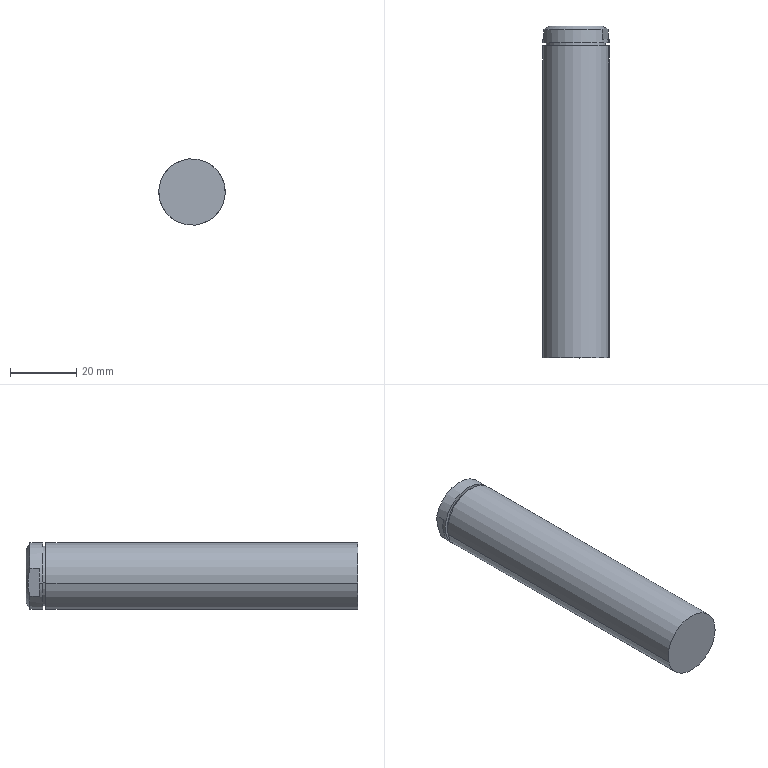Component | SolidWorks | SDA50-80CylinderPiston-1 | 1 solid | 20 faces | box 20 x 100 x 20 mm | volume 29602 mm3 | cylinder 8 | plane 8 | cone 4 | commonest cylinder face diameters 20 x4 18 x2 8.8 x2
build123d program:
from build123d import *

# Parameters (mm, degrees)
SKETCH1_R                   = 10
BOSS_EXTRUDE1_DEPTH         = 100
CHAMFER1_SIZE               = 2
CHAMFER1_SIZE2              = 1.155
CUT_EXTRUDE2_DEPTH          = 4
M10X1_25_TAPPED_HOLE1_D     = 8.8
M10X1_25_TAPPED_HOLE1_DEPTH = 26.25
M10X1_25_TAPPED_HOLE1_TIP   = 2.644
SKETCH6_W                   = 1
SKETCH6_H                   = 1


with BuildPart() as part:
    # Sketch1 → Boss-Extrude1 (new body)
    with BuildSketch(Plane.XY):
        Circle(SKETCH1_R)
    extrude(amount=BOSS_EXTRUDE1_DEPTH)

    # Chamfer1
    chamfer1_edges = [part.edges().sort_by_distance(p)[0] for p in [
        (-10, 0, 0),
    ]]
    chamfer1_side = [part.faces().sort_by_distance(p)[0] for p in [
        (0, 0, 0),
    ]]
    chamfer(chamfer1_edges, length=CHAMFER1_SIZE, length2=CHAMFER1_SIZE2, reference=chamfer1_side[0])

    # Sketch3 → Cut-Extrude2 (cut)
    with BuildSketch(Plane(origin=(0, 0, 0), x_dir=(-1, 0, 0), z_dir=(0, 0, -1))):
        with BuildLine():
            Line((9, 4.359), (9, -4.359))
            ThreePointArc((9, -4.359), (10, 0), (9, 4.359))
        make_face()
        with BuildLine():
            Line((-9, 4.359), (-9, -4.359))
            ThreePointArc((-9, -4.359), (-10, 0), (-9, 4.359))
        make_face()
    extrude(amount=-CUT_EXTRUDE2_DEPTH, mode=Mode.SUBTRACT)

    # M10x1.25 Tapped Hole1
    with Locations(Plane(origin=(0, 0, 0), x_dir=(-1, 0, 0), z_dir=(0, 0, -1))):
        with Locations((0, 0)):
            Hole(M10X1_25_TAPPED_HOLE1_D / 2, depth=M10X1_25_TAPPED_HOLE1_DEPTH)
            with Locations((0, 0, -(M10X1_25_TAPPED_HOLE1_DEPTH + M10X1_25_TAPPED_HOLE1_TIP / 2))):  # 118° drill point
                Cone(0, M10X1_25_TAPPED_HOLE1_D / 2, M10X1_25_TAPPED_HOLE1_TIP, mode=Mode.SUBTRACT)

    # Sketch6 → Cut-Revolve3 (revolve, cut)
    with BuildSketch(Plane(origin=(0, 0, 0), x_dir=(1, 0, 0), z_dir=(0, 1, 0))):
        with Locations((-9.5, -5.5)):
            Rectangle(SKETCH6_W, SKETCH6_H)
    revolve(axis=Axis((0, 0, 0), (0, 0, 1)), mode=Mode.SUBTRACT)


solid = part.part

# Placed as in the assembly
solid = solid.moved(Location((-29.507, -49.411, 430.5), (90, 0, 12.223)))
STEP:
#1=CARTESIAN_POINT('',(-0.7769,-5.882,17.032));
#2=VERTEX_POINT('',#1);
#3=CARTESIAN_POINT('',(-1.546,-5.882,16.865));
#4=VERTEX_POINT('',#3);
#5=CARTESIAN_POINT('',(-1.162,-5.882,16.949));
#6=DIRECTION('',(0.,-1.,0.));
#7=DIRECTION('',(0.9773,0.,0.2117));
#8=AXIS2_PLACEMENT_3D('',#5,#6,#7);
#9=CIRCLE('',#8,0.3937);
#10=EDGE_CURVE('',#2,#4,#9,.T.);
#11=ORIENTED_EDGE('',*,*,#10,.F.);
#12=CARTESIAN_POINT('',(-0.7769,-2.182,17.032));
#13=VERTEX_POINT('',#12);
#14=CARTESIAN_POINT('',(-0.7769,-5.882,17.032));
#15=DIRECTION('',(-0.,1.,-0.));
#16=VECTOR('',#15,39.37);
#17=LINE('',#14,#16);
#18=EDGE_CURVE('',#2,#13,#17,.T.);
#19=ORIENTED_EDGE('',*,*,#18,.T.);
#20=CARTESIAN_POINT('',(-1.546,-2.182,16.865));
#21=VERTEX_POINT('',#20);
#22=CARTESIAN_POINT('',(-1.162,-2.182,16.949));
#23=DIRECTION('',(-0.,1.,-0.));
#24=DIRECTION('',(-0.9773,0.,-0.2117));
#25=AXIS2_PLACEMENT_3D('',#22,#23,#24);
#26=CIRCLE('',#25,0.3937);
#27=EDGE_CURVE('',#21,#13,#26,.T.);
#28=ORIENTED_EDGE('',*,*,#27,.F.);
#29=CARTESIAN_POINT('',(-1.546,-5.882,16.865));
#30=DIRECTION('',(-0.,1.,-0.));
#31=VECTOR('',#30,39.37);
#32=LINE('',#29,#31);
#33=EDGE_CURVE('',#4,#21,#32,.T.);
#34=ORIENTED_EDGE('',*,*,#33,.F.);
#35=EDGE_LOOP('',(#11,#19,#28,#34));
#36=FACE_OUTER_BOUND('',#35,.T.);
#37=CARTESIAN_POINT('',(-1.162,-5.882,16.949));
#38=DIRECTION('',(-0.,1.,-0.));
#39=DIRECTION('',(-0.9773,0.,-0.2117));
#40=AXIS2_PLACEMENT_3D('',#37,#38,#39);
#41=CYLINDRICAL_SURFACE('',#40,0.3937);
#42=ADVANCED_FACE('',(#36),#41,.T.);
#43=CARTESIAN_POINT('',(-1.508,-2.182,16.874));
#44=VERTEX_POINT('',#43);
#45=CARTESIAN_POINT('',(-0.8154,-2.182,17.024));
#46=VERTEX_POINT('',#45);
#47=CARTESIAN_POINT('',(-1.162,-2.182,16.949));
#48=DIRECTION('',(-0.,1.,-0.));
#49=DIRECTION('',(-0.9773,0.,-0.2117));
#50=AXIS2_PLACEMENT_3D('',#47,#48,#49);
#51=CIRCLE('',#50,0.3543);
#52=EDGE_CURVE('',#44,#46,#51,.T.);
#53=ORIENTED_EDGE('',*,*,#52,.T.);
#54=CARTESIAN_POINT('',(-0.8154,-2.142,17.024));
#55=VERTEX_POINT('',#54);
#56=CARTESIAN_POINT('',(-0.8154,-1.945,17.024));
#57=DIRECTION('',(-0.,1.,-0.));
#58=VECTOR('',#57,39.37);
#59=LINE('',#56,#58);
#60=EDGE_CURVE('',#46,#55,#59,.T.);
#61=ORIENTED_EDGE('',*,*,#60,.T.);
#62=CARTESIAN_POINT('',(-1.508,-2.142,16.874));
#63=VERTEX_POINT('',#62);
#64=CARTESIAN_POINT('',(-1.162,-2.142,16.949));
#65=DIRECTION('',(-0.,1.,-0.));
#66=DIRECTION('',(-0.9773,0.,-0.2117));
#67=AXIS2_PLACEMENT_3D('',#64,#65,#66);
#68=CIRCLE('',#67,0.3543);
#69=EDGE_CURVE('',#63,#55,#68,.T.);
#70=ORIENTED_EDGE('',*,*,#69,.F.);
#71=CARTESIAN_POINT('',(-1.508,-1.945,16.874));
#72=DIRECTION('',(-0.,1.,-0.));
#73=VECTOR('',#72,39.37);
#74=LINE('',#71,#73);
#75=EDGE_CURVE('',#44,#63,#74,.T.);
#76=ORIENTED_EDGE('',*,*,#75,.F.);
#77=EDGE_LOOP('',(#53,#61,#70,#76));
#78=FACE_OUTER_BOUND('',#77,.T.);
#79=CARTESIAN_POINT('',(-1.162,-1.945,16.949));
#80=DIRECTION('',(-0.,1.,-0.));
#81=DIRECTION('',(-0.9773,0.,-0.2117));
#82=AXIS2_PLACEMENT_3D('',#79,#80,#81);
#83=CYLINDRICAL_SURFACE('',#82,0.3543);
#84=ADVANCED_FACE('',(#78),#83,.T.);
#85=CARTESIAN_POINT('',(-0.9924,-2.979,16.985));
#86=VERTEX_POINT('',#85);
#87=CARTESIAN_POINT('',(-1.331,-2.979,16.912));
#88=VERTEX_POINT('',#87);
#89=CARTESIAN_POINT('',(-1.162,-2.979,16.949));
#90=DIRECTION('',(-0.,1.,-0.));
#91=DIRECTION('',(-0.9773,0.,-0.2117));
#92=AXIS2_PLACEMENT_3D('',#89,#90,#91);
#93=CIRCLE('',#92,0.1732);
#94=EDGE_CURVE('',#86,#88,#93,.T.);
#95=ORIENTED_EDGE('',*,*,#94,.F.);
#96=CARTESIAN_POINT('',(-0.9924,-1.945,16.985));
#97=VERTEX_POINT('',#96);
#98=CARTESIAN_POINT('',(-0.9924,-1.945,16.985));
#99=DIRECTION('',(-0.,1.,-0.));
#100=VECTOR('',#99,39.37);
#101=LINE('',#98,#100);
#102=EDGE_CURVE('',#86,#97,#101,.T.);
#103=ORIENTED_EDGE('',*,*,#102,.T.);
#104=CARTESIAN_POINT('',(-1.331,-1.945,16.912));
#105=VERTEX_POINT('',#104);
#106=CARTESIAN_POINT('',(-1.162,-1.945,16.949));
#107=DIRECTION('',(-0.,1.,-0.));
#108=DIRECTION('',(-0.9773,0.,-0.2117));
#109=AXIS2_PLACEMENT_3D('',#106,#107,#108);
#110=CIRCLE('',#109,0.1732);
#111=EDGE_CURVE('',#97,#105,#110,.T.);
#112=ORIENTED_EDGE('',*,*,#111,.T.);
#113=CARTESIAN_POINT('',(-1.331,-1.945,16.912));
#114=DIRECTION('',(-0.,1.,-0.));
#115=VECTOR('',#114,39.37);
#116=LINE('',#113,#115);
#117=EDGE_CURVE('',#88,#105,#116,.T.);
#118=ORIENTED_EDGE('',*,*,#117,.F.);
#119=EDGE_LOOP('',(#95,#103,#112,#118));
#120=FACE_OUTER_BOUND('',#119,.T.);
#121=CARTESIAN_POINT('',(-1.162,-1.945,16.949));
#122=DIRECTION('',(-0.,1.,-0.));
#123=DIRECTION('',(-0.9773,0.,-0.2117));
#124=AXIS2_PLACEMENT_3D('',#121,#122,#123);
#125=CYLINDRICAL_SURFACE('',#124,0.1732);
#126=ADVANCED_FACE('',(#120),#125,.F.);
#127=CARTESIAN_POINT('',(-1.162,-3.083,16.949));
#128=VERTEX_POINT('',#127);
#129=CARTESIAN_POINT('',(-1.331,-2.979,16.912));
#130=DIRECTION('',(-0.8377,0.515,-0.1815));
#131=VECTOR('',#130,39.37);
#132=LINE('',#129,#131);
#133=EDGE_CURVE('',#128,#88,#132,.T.);
#134=ORIENTED_EDGE('',*,*,#133,.F.);
#135=CARTESIAN_POINT('',(-0.9924,-2.979,16.985));
#136=DIRECTION('',(0.8377,0.515,0.1815));
#137=VECTOR('',#136,39.37);
#138=LINE('',#135,#137);
#139=EDGE_CURVE('',#128,#86,#138,.T.);
#140=ORIENTED_EDGE('',*,*,#139,.T.);
#141=ORIENTED_EDGE('',*,*,#94,.T.);
#142=EDGE_LOOP('',(#134,#140,#141));
#143=FACE_OUTER_BOUND('',#142,.T.);
#144=CARTESIAN_POINT('',(-1.162,-2.979,16.949));
#145=DIRECTION('',(-0.,1.,-0.));
#146=DIRECTION('',(-0.9773,0.,-0.2117));
#147=AXIS2_PLACEMENT_3D('',#144,#145,#146);
#148=CONICAL_SURFACE('',#147,0.1732,1.03);
#149=ADVANCED_FACE('',(#143),#148,.F.);
#150=CARTESIAN_POINT('',(-1.469,-1.945,16.882));
#151=VERTEX_POINT('',#150);
#152=CARTESIAN_POINT('',(-0.8539,-1.945,17.016));
#153=VERTEX_POINT('',#152);
#154=CARTESIAN_POINT('',(-1.162,-1.945,16.949));
#155=DIRECTION('',(-0.,1.,-0.));
#156=DIRECTION('',(0.9773,0.,0.2117));
#157=AXIS2_PLACEMENT_3D('',#154,#155,#156);
#158=CIRCLE('',#157,0.315);
#159=EDGE_CURVE('',#151,#153,#158,.T.);
#160=ORIENTED_EDGE('',*,*,#159,.F.);
#161=CARTESIAN_POINT('',(-1.508,-1.968,16.874));
#162=VERTEX_POINT('',#161);
#163=CARTESIAN_POINT('',(-1.546,-1.991,16.865));
#164=DIRECTION('',(-0.8464,-0.5,-0.1834));
#165=VECTOR('',#164,39.37);
#166=LINE('',#163,#165);
#167=EDGE_CURVE('',#151,#162,#166,.T.);
#168=ORIENTED_EDGE('',*,*,#167,.T.);
#169=CARTESIAN_POINT('',(-1.544,-1.991,17.042));
#170=VERTEX_POINT('',#169);
#171=CARTESIAN_POINT('',(-1.544,-1.991,17.042));
#172=CARTESIAN_POINT('',(-1.538,-1.984,17.014));
#173=CARTESIAN_POINT('',(-1.532,-1.978,16.987));
#174=CARTESIAN_POINT('',(-1.523,-1.972,16.944));
#175=CARTESIAN_POINT('',(-1.52,-1.971,16.93));
#176=CARTESIAN_POINT('',(-1.514,-1.969,16.902));
#177=CARTESIAN_POINT('',(-1.511,-1.968,16.888));
#178=CARTESIAN_POINT('',(-1.508,-1.968,16.874));
#179=B_SPLINE_CURVE_WITH_KNOTS('',3,(#171,#172,#173,#174,#175,#176,#177,#178),.UNSPECIFIED.,.F.,.F.,(4,2,2,4),(0.005779,0.007969,0.009064,0.01016),.UNSPECIFIED.);
#180=EDGE_CURVE('',#170,#162,#179,.T.);
#181=ORIENTED_EDGE('',*,*,#180,.F.);
#182=CARTESIAN_POINT('',(-0.8517,-1.991,17.192));
#183=VERTEX_POINT('',#182);
#184=CARTESIAN_POINT('',(-1.162,-1.991,16.949));
#185=DIRECTION('',(0.,-1.,0.));
#186=DIRECTION('',(0.9773,0.,0.2117));
#187=AXIS2_PLACEMENT_3D('',#184,#185,#186);
#188=CIRCLE('',#187,0.3937);
#189=EDGE_CURVE('',#183,#170,#188,.T.);
#190=ORIENTED_EDGE('',*,*,#189,.F.);
#191=CARTESIAN_POINT('',(-0.8154,-1.968,17.024));
#192=VERTEX_POINT('',#191);
#193=CARTESIAN_POINT('',(-0.8154,-1.968,17.024));
#194=CARTESIAN_POINT('',(-0.8184,-1.968,17.038));
#195=CARTESIAN_POINT('',(-0.8215,-1.969,17.052));
#196=CARTESIAN_POINT('',(-0.8276,-1.971,17.08));
#197=CARTESIAN_POINT('',(-0.8307,-1.972,17.094));
#198=CARTESIAN_POINT('',(-0.8398,-1.978,17.137));
#199=CARTESIAN_POINT('',(-0.8458,-1.984,17.164));
#200=CARTESIAN_POINT('',(-0.8517,-1.991,17.192));
#201=B_SPLINE_CURVE_WITH_KNOTS('',3,(#193,#194,#195,#196,#197,#198,#199,#200),.UNSPECIFIED.,.F.,.F.,(4,2,2,4),(0.01291,0.014,0.0151,0.01729),.UNSPECIFIED.);
#202=EDGE_CURVE('',#192,#183,#201,.T.);
#203=ORIENTED_EDGE('',*,*,#202,.F.);
#204=CARTESIAN_POINT('',(-0.7769,-1.991,17.032));
#205=DIRECTION('',(0.8464,-0.5,0.1834));
#206=VECTOR('',#205,39.37);
#207=LINE('',#204,#206);
#208=EDGE_CURVE('',#153,#192,#207,.T.);
#209=ORIENTED_EDGE('',*,*,#208,.F.);
#210=EDGE_LOOP('',(#160,#168,#181,#190,#203,#209));
#211=FACE_OUTER_BOUND('',#210,.T.);
#212=CARTESIAN_POINT('',(-1.162,-1.991,16.949));
#213=DIRECTION('',(0.,-1.,0.));
#214=DIRECTION('',(0.9773,0.,0.2117));
#215=AXIS2_PLACEMENT_3D('',#212,#213,#214);
#216=CONICAL_SURFACE('',#215,0.3937,1.047);
#217=ADVANCED_FACE('',(#211),#216,.T.);
#218=CARTESIAN_POINT('',(-1.546,-2.142,16.865));
#219=VERTEX_POINT('',#218);
#220=CARTESIAN_POINT('',(-0.7769,-2.142,17.032));
#221=VERTEX_POINT('',#220);
#222=CARTESIAN_POINT('',(-1.162,-2.142,16.949));
#223=DIRECTION('',(-0.,1.,-0.));
#224=DIRECTION('',(-0.9773,0.,-0.2117));
#225=AXIS2_PLACEMENT_3D('',#222,#223,#224);
#226=CIRCLE('',#225,0.3937);
#227=EDGE_CURVE('',#219,#221,#226,.T.);
#228=ORIENTED_EDGE('',*,*,#227,.T.);
#229=CARTESIAN_POINT('',(-0.7769,-2.103,17.032));
#230=VERTEX_POINT('',#229);
#231=CARTESIAN_POINT('',(-0.7769,-5.882,17.032));
#232=DIRECTION('',(-0.,1.,-0.));
#233=VECTOR('',#232,39.37);
#234=LINE('',#231,#233);
#235=EDGE_CURVE('',#221,#230,#234,.T.);
#236=ORIENTED_EDGE('',*,*,#235,.T.);
#237=CARTESIAN_POINT('',(-0.8517,-2.103,17.192));
#238=VERTEX_POINT('',#237);
#239=CARTESIAN_POINT('',(-1.162,-2.103,16.949));
#240=DIRECTION('',(-0.,1.,-0.));
#241=DIRECTION('',(-0.9773,0.,-0.2117));
#242=AXIS2_PLACEMENT_3D('',#239,#240,#241);
#243=CIRCLE('',#242,0.3937);
#244=EDGE_CURVE('',#238,#230,#243,.T.);
#245=ORIENTED_EDGE('',*,*,#244,.F.);
#246=CARTESIAN_POINT('',(-0.8517,-2.103,17.192));
#247=DIRECTION('',(-0.,1.,-0.));
#248=VECTOR('',#247,39.37);
#249=LINE('',#246,#248);
#250=EDGE_CURVE('',#238,#183,#249,.T.);
#251=ORIENTED_EDGE('',*,*,#250,.T.);
#252=ORIENTED_EDGE('',*,*,#189,.T.);
#253=CARTESIAN_POINT('',(-1.544,-2.103,17.042));
#254=VERTEX_POINT('',#253);
#255=CARTESIAN_POINT('',(-1.544,-2.103,17.042));
#256=DIRECTION('',(-0.,1.,-0.));
#257=VECTOR('',#256,39.37);
#258=LINE('',#255,#257);
#259=EDGE_CURVE('',#254,#170,#258,.T.);
#260=ORIENTED_EDGE('',*,*,#259,.F.);
#261=CARTESIAN_POINT('',(-1.546,-2.103,16.865));
#262=VERTEX_POINT('',#261);
#263=CARTESIAN_POINT('',(-1.162,-2.103,16.949));
#264=DIRECTION('',(-0.,1.,-0.));
#265=DIRECTION('',(-0.9773,0.,-0.2117));
#266=AXIS2_PLACEMENT_3D('',#263,#264,#265);
#267=CIRCLE('',#266,0.3937);
#268=EDGE_CURVE('',#262,#254,#267,.T.);
#269=ORIENTED_EDGE('',*,*,#268,.F.);
#270=CARTESIAN_POINT('',(-1.546,-5.882,16.865));
#271=DIRECTION('',(-0.,1.,-0.));
#272=VECTOR('',#271,39.37);
#273=LINE('',#270,#272);
#274=EDGE_CURVE('',#219,#262,#273,.T.);
#275=ORIENTED_EDGE('',*,*,#274,.F.);
#276=EDGE_LOOP('',(#228,#236,#245,#251,#252,#260,#269,#275));
#277=FACE_OUTER_BOUND('',#276,.T.);
#278=CARTESIAN_POINT('',(-1.162,-5.882,16.949));
#279=DIRECTION('',(-0.,1.,-0.));
#280=DIRECTION('',(-0.9773,0.,-0.2117));
#281=AXIS2_PLACEMENT_3D('',#278,#279,#280);
#282=CYLINDRICAL_SURFACE('',#281,0.3937);
#283=ADVANCED_FACE('',(#277),#282,.T.);
#284=ORIENTED_EDGE('',*,*,#235,.F.);
#285=CARTESIAN_POINT('',(-1.162,-2.142,16.949));
#286=DIRECTION('',(-0.,1.,-0.));
#287=DIRECTION('',(-0.9773,0.,-0.2117));
#288=AXIS2_PLACEMENT_3D('',#285,#286,#287);
#289=CIRCLE('',#288,0.3937);
#290=EDGE_CURVE('',#221,#219,#289,.T.);
#291=ORIENTED_EDGE('',*,*,#290,.T.);
#292=ORIENTED_EDGE('',*,*,#274,.T.);
#293=CARTESIAN_POINT('',(-1.472,-2.103,16.706));
#294=VERTEX_POINT('',#293);
#295=CARTESIAN_POINT('',(-1.162,-2.103,16.949));
#296=DIRECTION('',(-0.,1.,-0.));
#297=DIRECTION('',(-0.9773,0.,-0.2117));
#298=AXIS2_PLACEMENT_3D('',#295,#296,#297);
#299=CIRCLE('',#298,0.3937);
#300=EDGE_CURVE('',#294,#262,#299,.T.);
#301=ORIENTED_EDGE('',*,*,#300,.F.);
#302=CARTESIAN_POINT('',(-1.472,-1.991,16.706));
#303=VERTEX_POINT('',#302);
#304=CARTESIAN_POINT('',(-1.472,-2.103,16.706));
#305=DIRECTION('',(-0.,1.,-0.));
#306=VECTOR('',#305,39.37);
#307=LINE('',#304,#306);
#308=EDGE_CURVE('',#294,#303,#307,.T.);
#309=ORIENTED_EDGE('',*,*,#308,.T.);
#310=CARTESIAN_POINT('',(-0.779,-1.991,16.856));
#311=VERTEX_POINT('',#310);
#312=CARTESIAN_POINT('',(-1.162,-1.991,16.949));
#313=DIRECTION('',(0.,-1.,0.));
#314=DIRECTION('',(0.9773,0.,0.2117));
#315=AXIS2_PLACEMENT_3D('',#312,#313,#314);
#316=CIRCLE('',#315,0.3937);
#317=EDGE_CURVE('',#303,#311,#316,.T.);
#318=ORIENTED_EDGE('',*,*,#317,.T.);
#319=CARTESIAN_POINT('',(-0.779,-2.103,16.856));
#320=VERTEX_POINT('',#319);
#321=CARTESIAN_POINT('',(-0.779,-2.103,16.856));
#322=DIRECTION('',(-0.,1.,-0.));
#323=VECTOR('',#322,39.37);
#324=LINE('',#321,#323);
#325=EDGE_CURVE('',#320,#311,#324,.T.);
#326=ORIENTED_EDGE('',*,*,#325,.F.);
#327=CARTESIAN_POINT('',(-1.162,-2.103,16.949));
#328=DIRECTION('',(-0.,1.,-0.));
#329=DIRECTION('',(-0.9773,0.,-0.2117));
#330=AXIS2_PLACEMENT_3D('',#327,#328,#329);
#331=CIRCLE('',#330,0.3937);
#332=EDGE_CURVE('',#230,#320,#331,.T.);
#333=ORIENTED_EDGE('',*,*,#332,.F.);
#334=EDGE_LOOP('',(#284,#291,#292,#301,#309,#318,#326,#333));
#335=FACE_OUTER_BOUND('',#334,.T.);
#336=CARTESIAN_POINT('',(-1.162,-5.882,16.949));
#337=DIRECTION('',(-0.,1.,-0.));
#338=DIRECTION('',(-0.9773,0.,-0.2117));
#339=AXIS2_PLACEMENT_3D('',#336,#337,#338);
#340=CYLINDRICAL_SURFACE('',#339,0.3937);
#341=ADVANCED_FACE('',(#335),#340,.T.);
#342=CARTESIAN_POINT('',(-1.162,-1.945,16.949));
#343=DIRECTION('',(-0.,1.,-0.));
#344=DIRECTION('',(-0.9773,0.,-0.2117));
#345=AXIS2_PLACEMENT_3D('',#342,#343,#344);
#346=CIRCLE('',#345,0.1732);
#347=EDGE_CURVE('',#105,#97,#346,.T.);
#348=ORIENTED_EDGE('',*,*,#347,.F.);
#349=ORIENTED_EDGE('',*,*,#111,.F.);
#350=EDGE_LOOP('',(#348,#349));
#351=FACE_BOUND('',#350,.T.);
#352=CARTESIAN_POINT('',(-1.162,-1.945,16.949));
#353=DIRECTION('',(-0.,1.,-0.));
#354=DIRECTION('',(0.9773,0.,0.2117));
#355=AXIS2_PLACEMENT_3D('',#352,#353,#354);
#356=CIRCLE('',#355,0.315);
#357=EDGE_CURVE('',#153,#151,#356,.T.);
#358=ORIENTED_EDGE('',*,*,#357,.T.);
#359=ORIENTED_EDGE('',*,*,#159,.T.);
#360=EDGE_LOOP('',(#358,#359));
#361=FACE_OUTER_BOUND('',#360,.T.);
#362=CARTESIAN_POINT('',(-1.162,-1.945,16.949));
#363=DIRECTION('',(0.,-1.,0.));
#364=DIRECTION('',(0.9773,0.,0.2117));
#365=AXIS2_PLACEMENT_3D('',#362,#363,#364);
#366=PLANE('',#365);
#367=ADVANCED_FACE('',(#351,#361),#366,.F.);
#368=ORIENTED_EDGE('',*,*,#167,.F.);
#369=ORIENTED_EDGE('',*,*,#357,.F.);
#370=ORIENTED_EDGE('',*,*,#208,.T.);
#371=CARTESIAN_POINT('',(-0.779,-1.991,16.856));
#372=CARTESIAN_POINT('',(-0.785,-1.984,16.884));
#373=CARTESIAN_POINT('',(-0.7911,-1.978,16.912));
#374=CARTESIAN_POINT('',(-0.8032,-1.97,16.968));
#375=CARTESIAN_POINT('',(-0.8093,-1.968,16.996));
#376=CARTESIAN_POINT('',(-0.8154,-1.968,17.024));
#377=B_SPLINE_CURVE_WITH_KNOTS('',3,(#371,#372,#373,#374,#375,#376),.UNSPECIFIED.,.F.,.F.,(4,2,4),(0.008519,0.01071,0.01291),.UNSPECIFIED.);
#378=EDGE_CURVE('',#311,#192,#377,.T.);
#379=ORIENTED_EDGE('',*,*,#378,.F.);
#380=ORIENTED_EDGE('',*,*,#317,.F.);
#381=CARTESIAN_POINT('',(-1.508,-1.968,16.874));
#382=CARTESIAN_POINT('',(-1.502,-1.968,16.846));
#383=CARTESIAN_POINT('',(-1.496,-1.97,16.818));
#384=CARTESIAN_POINT('',(-1.484,-1.978,16.762));
#385=CARTESIAN_POINT('',(-1.478,-1.984,16.733));
#386=CARTESIAN_POINT('',(-1.472,-1.991,16.706));
#387=B_SPLINE_CURVE_WITH_KNOTS('',3,(#381,#382,#383,#384,#385,#386),.UNSPECIFIED.,.F.,.F.,(4,2,4),(0.01016,0.01235,0.01454),.UNSPECIFIED.);
#388=EDGE_CURVE('',#162,#303,#387,.T.);
#389=ORIENTED_EDGE('',*,*,#388,.F.);
#390=EDGE_LOOP('',(#368,#369,#370,#379,#380,#389));
#391=FACE_OUTER_BOUND('',#390,.T.);
#392=CARTESIAN_POINT('',(-1.162,-1.991,16.949));
#393=DIRECTION('',(0.,-1.,0.));
#394=DIRECTION('',(0.9773,0.,0.2117));
#395=AXIS2_PLACEMENT_3D('',#392,#393,#394);
#396=CONICAL_SURFACE('',#395,0.3937,1.047);
#397=ADVANCED_FACE('',(#391),#396,.T.);
#398=ORIENTED_EDGE('',*,*,#378,.T.);
#399=ORIENTED_EDGE('',*,*,#202,.T.);
#400=ORIENTED_EDGE('',*,*,#250,.F.);
#401=CARTESIAN_POINT('',(-0.8517,-2.103,17.192));
#402=DIRECTION('',(-0.2117,0.,0.9773));
#403=VECTOR('',#402,39.37);
#404=LINE('',#401,#403);
#405=EDGE_CURVE('',#320,#238,#404,.T.);
#406=ORIENTED_EDGE('',*,*,#405,.F.);
#407=ORIENTED_EDGE('',*,*,#325,.T.);
#408=EDGE_LOOP('',(#398,#399,#400,#406,#407));
#409=FACE_OUTER_BOUND('',#408,.T.);
#410=CARTESIAN_POINT('',(-0.8517,-2.103,17.192));
#411=DIRECTION('',(-0.9773,-0.,-0.2117));
#412=DIRECTION('',(0.,-1.,0.));
#413=AXIS2_PLACEMENT_3D('',#410,#411,#412);
#414=PLANE('',#413);
#415=ADVANCED_FACE('',(#409),#414,.F.);
#416=ORIENTED_EDGE('',*,*,#244,.T.);
#417=ORIENTED_EDGE('',*,*,#332,.T.);
#418=ORIENTED_EDGE('',*,*,#405,.T.);
#419=EDGE_LOOP('',(#416,#417,#418));
#420=FACE_OUTER_BOUND('',#419,.T.);
#421=CARTESIAN_POINT('',(-1.162,-2.103,16.949));
#422=DIRECTION('',(-0.,1.,-0.));
#423=DIRECTION('',(-0.9773,-0.,-0.2117));
#424=AXIS2_PLACEMENT_3D('',#421,#422,#423);
#425=PLANE('',#424);
#426=ADVANCED_FACE('',(#420),#425,.T.);
#427=ORIENTED_EDGE('',*,*,#180,.T.);
#428=ORIENTED_EDGE('',*,*,#388,.T.);
#429=ORIENTED_EDGE('',*,*,#308,.F.);
#430=CARTESIAN_POINT('',(-1.544,-2.103,17.042));
#431=DIRECTION('',(0.2117,-0.,-0.9773));
#432=VECTOR('',#431,39.37);
#433=LINE('',#430,#432);
#434=EDGE_CURVE('',#254,#294,#433,.T.);
#435=ORIENTED_EDGE('',*,*,#434,.F.);
#436=ORIENTED_EDGE('',*,*,#259,.T.);
#437=EDGE_LOOP('',(#427,#428,#429,#435,#436));
#438=FACE_OUTER_BOUND('',#437,.T.);
#439=CARTESIAN_POINT('',(-1.544,-2.103,17.042));
#440=DIRECTION('',(0.9773,0.,0.2117));
#441=DIRECTION('',(-0.,1.,-0.));
#442=AXIS2_PLACEMENT_3D('',#439,#440,#441);
#443=PLANE('',#442);
#444=ADVANCED_FACE('',(#438),#443,.F.);
#445=ORIENTED_EDGE('',*,*,#300,.T.);
#446=ORIENTED_EDGE('',*,*,#268,.T.);
#447=ORIENTED_EDGE('',*,*,#434,.T.);
#448=EDGE_LOOP('',(#445,#446,#447));
#449=FACE_OUTER_BOUND('',#448,.T.);
#450=CARTESIAN_POINT('',(-1.162,-2.103,16.949));
#451=DIRECTION('',(-0.,1.,-0.));
#452=DIRECTION('',(-0.9773,-0.,-0.2117));
#453=AXIS2_PLACEMENT_3D('',#450,#451,#452);
#454=PLANE('',#453);
#455=ADVANCED_FACE('',(#449),#454,.T.);
#456=ORIENTED_EDGE('',*,*,#139,.F.);
#457=ORIENTED_EDGE('',*,*,#133,.T.);
#458=CARTESIAN_POINT('',(-1.162,-2.979,16.949));
#459=DIRECTION('',(-0.,1.,-0.));
#460=DIRECTION('',(-0.9773,0.,-0.2117));
#461=AXIS2_PLACEMENT_3D('',#458,#459,#460);
#462=CIRCLE('',#461,0.1732);
#463=EDGE_CURVE('',#88,#86,#462,.T.);
#464=ORIENTED_EDGE('',*,*,#463,.T.);
#465=EDGE_LOOP('',(#456,#457,#464));
#466=FACE_OUTER_BOUND('',#465,.T.);
#467=CARTESIAN_POINT('',(-1.162,-2.979,16.949));
#468=DIRECTION('',(-0.,1.,-0.));
#469=DIRECTION('',(-0.9773,0.,-0.2117));
#470=AXIS2_PLACEMENT_3D('',#467,#468,#469);
#471=CONICAL_SURFACE('',#470,0.1732,1.03);
#472=ADVANCED_FACE('',(#466),#471,.F.);
#473=ORIENTED_EDGE('',*,*,#102,.F.);
#474=ORIENTED_EDGE('',*,*,#463,.F.);
#475=ORIENTED_EDGE('',*,*,#117,.T.);
#476=ORIENTED_EDGE('',*,*,#347,.T.);
#477=EDGE_LOOP('',(#473,#474,#475,#476));
#478=FACE_OUTER_BOUND('',#477,.T.);
#479=CARTESIAN_POINT('',(-1.162,-1.945,16.949));
#480=DIRECTION('',(-0.,1.,-0.));
#481=DIRECTION('',(-0.9773,0.,-0.2117));
#482=AXIS2_PLACEMENT_3D('',#479,#480,#481);
#483=CYLINDRICAL_SURFACE('',#482,0.1732);
#484=ADVANCED_FACE('',(#478),#483,.F.);
#485=ORIENTED_EDGE('',*,*,#60,.F.);
#486=CARTESIAN_POINT('',(-1.162,-2.182,16.949));
#487=DIRECTION('',(-0.,1.,-0.));
#488=DIRECTION('',(-0.9773,0.,-0.2117));
#489=AXIS2_PLACEMENT_3D('',#486,#487,#488);
#490=CIRCLE('',#489,0.3543);
#491=EDGE_CURVE('',#46,#44,#490,.T.);
#492=ORIENTED_EDGE('',*,*,#491,.T.);
#493=ORIENTED_EDGE('',*,*,#75,.T.);
#494=CARTESIAN_POINT('',(-1.162,-2.142,16.949));
#495=DIRECTION('',(-0.,1.,-0.));
#496=DIRECTION('',(-0.9773,0.,-0.2117));
#497=AXIS2_PLACEMENT_3D('',#494,#495,#496);
#498=CIRCLE('',#497,0.3543);
#499=EDGE_CURVE('',#55,#63,#498,.T.);
#500=ORIENTED_EDGE('',*,*,#499,.F.);
#501=EDGE_LOOP('',(#485,#492,#493,#500));
#502=FACE_OUTER_BOUND('',#501,.T.);
#503=CARTESIAN_POINT('',(-1.162,-1.945,16.949));
#504=DIRECTION('',(-0.,1.,-0.));
#505=DIRECTION('',(-0.9773,0.,-0.2117));
#506=AXIS2_PLACEMENT_3D('',#503,#504,#505);
#507=CYLINDRICAL_SURFACE('',#506,0.3543);
#508=ADVANCED_FACE('',(#502),#507,.T.);
#509=ORIENTED_EDGE('',*,*,#52,.F.);
#510=ORIENTED_EDGE('',*,*,#491,.F.);
#511=EDGE_LOOP('',(#509,#510));
#512=FACE_BOUND('',#511,.T.);
#513=ORIENTED_EDGE('',*,*,#27,.T.);
#514=CARTESIAN_POINT('',(-1.162,-2.182,16.949));
#515=DIRECTION('',(-0.,1.,-0.));
#516=DIRECTION('',(-0.9773,0.,-0.2117));
#517=AXIS2_PLACEMENT_3D('',#514,#515,#516);
#518=CIRCLE('',#517,0.3937);
#519=EDGE_CURVE('',#13,#21,#518,.T.);
#520=ORIENTED_EDGE('',*,*,#519,.T.);
#521=EDGE_LOOP('',(#513,#520));
#522=FACE_OUTER_BOUND('',#521,.T.);
#523=CARTESIAN_POINT('',(-1.508,-2.182,16.874));
#524=DIRECTION('',(0.,-1.,0.));
#525=DIRECTION('',(0.9773,0.,0.2117));
#526=AXIS2_PLACEMENT_3D('',#523,#524,#525);
#527=PLANE('',#526);
#528=ADVANCED_FACE('',(#512,#522),#527,.F.);
#529=ORIENTED_EDGE('',*,*,#227,.F.);
#530=ORIENTED_EDGE('',*,*,#290,.F.);
#531=EDGE_LOOP('',(#529,#530));
#532=FACE_OUTER_BOUND('',#531,.T.);
#533=ORIENTED_EDGE('',*,*,#69,.T.);
#534=ORIENTED_EDGE('',*,*,#499,.T.);
#535=EDGE_LOOP('',(#533,#534));
#536=FACE_BOUND('',#535,.T.);
#537=CARTESIAN_POINT('',(-1.508,-2.142,16.874));
#538=DIRECTION('',(-0.,1.,-0.));
#539=DIRECTION('',(-0.9773,-0.,-0.2117));
#540=AXIS2_PLACEMENT_3D('',#537,#538,#539);
#541=PLANE('',#540);
#542=ADVANCED_FACE('',(#532,#536),#541,.F.);
#543=CARTESIAN_POINT('',(-1.162,-5.882,16.949));
#544=DIRECTION('',(0.,-1.,0.));
#545=DIRECTION('',(0.9773,0.,0.2117));
#546=AXIS2_PLACEMENT_3D('',#543,#544,#545);
#547=CIRCLE('',#546,0.3937);
#548=EDGE_CURVE('',#4,#2,#547,.T.);
#549=ORIENTED_EDGE('',*,*,#548,.T.);
#550=ORIENTED_EDGE('',*,*,#10,.T.);
#551=EDGE_LOOP('',(#549,#550));
#552=FACE_OUTER_BOUND('',#551,.T.);
#553=CARTESIAN_POINT('',(-1.162,-5.882,16.949));
#554=DIRECTION('',(0.,-1.,0.));
#555=DIRECTION('',(0.9773,0.,0.2117));
#556=AXIS2_PLACEMENT_3D('',#553,#554,#555);
#557=PLANE('',#556);
#558=ADVANCED_FACE('',(#552),#557,.T.);
#559=ORIENTED_EDGE('',*,*,#18,.F.);
#560=ORIENTED_EDGE('',*,*,#548,.F.);
#561=ORIENTED_EDGE('',*,*,#33,.T.);
#562=ORIENTED_EDGE('',*,*,#519,.F.);
#563=EDGE_LOOP('',(#559,#560,#561,#562));
#564=FACE_OUTER_BOUND('',#563,.T.);
#565=CARTESIAN_POINT('',(-1.162,-5.882,16.949));
#566=DIRECTION('',(-0.,1.,-0.));
#567=DIRECTION('',(-0.9773,0.,-0.2117));
#568=AXIS2_PLACEMENT_3D('',#565,#566,#567);
#569=CYLINDRICAL_SURFACE('',#568,0.3937);
#570=ADVANCED_FACE('',(#564),#569,.T.);
#571=CLOSED_SHELL('',(#42,#84,#126,#149,#217,#283,#341,#367,#397,#415,#426,#444,#455,#472,#484,#508,#528,#542,#558,#570));
#572=MANIFOLD_SOLID_BREP('',#571);
#573=CARTESIAN_POINT('',(0.,0.,0.));
#574=DIRECTION('',(0.,0.,1.));
#575=DIRECTION('',(1.,0.,0.));
#576=AXIS2_PLACEMENT_3D('',#573,#574,#575);
#577=(LENGTH_UNIT()NAMED_UNIT(*)SI_UNIT($,.METRE.));
#578=LENGTH_MEASURE_WITH_UNIT(LENGTH_MEASURE(0.0254),#577);
#579=DIMENSIONAL_EXPONENTS(1.,0.,0.,0.,0.,0.,0.);
#580=(CONVERSION_BASED_UNIT('',#578)LENGTH_UNIT()NAMED_UNIT(#579));
#581=UNCERTAINTY_MEASURE_WITH_UNIT(LENGTH_MEASURE(0.00001),#580,'','');
#582=(NAMED_UNIT(*)PLANE_ANGLE_UNIT()SI_UNIT($,.RADIAN.));
#583=(NAMED_UNIT(*)SI_UNIT($,.STERADIAN.)SOLID_ANGLE_UNIT());
#584=(GEOMETRIC_REPRESENTATION_CONTEXT(3)GLOBAL_UNCERTAINTY_ASSIGNED_CONTEXT((#581))GLOBAL_UNIT_ASSIGNED_CONTEXT((#580,#582,#583))REPRESENTATION_CONTEXT('',''));
#585=ADVANCED_BREP_SHAPE_REPRESENTATION('',(#572,#576),#584);
#586=COLOUR_RGB('',0.7922,0.8196,0.9333);
#587=FILL_AREA_STYLE_COLOUR('',#586);
#588=FILL_AREA_STYLE('',(#587));
#589=SURFACE_STYLE_FILL_AREA(#588);
#590=SURFACE_SIDE_STYLE('',(#589));
#591=SURFACE_STYLE_USAGE(.BOTH.,#590);
#592=PRESENTATION_STYLE_ASSIGNMENT((#591));
#593=STYLED_ITEM('',(#592),#572);
#594=(LENGTH_UNIT()NAMED_UNIT(*)SI_UNIT($,.METRE.));
#595=LENGTH_MEASURE_WITH_UNIT(LENGTH_MEASURE(0.0254),#594);
#596=DIMENSIONAL_EXPONENTS(1.,0.,0.,0.,0.,0.,0.);
#597=(CONVERSION_BASED_UNIT('',#595)LENGTH_UNIT()NAMED_UNIT(#596));
#598=UNCERTAINTY_MEASURE_WITH_UNIT(LENGTH_MEASURE(0.00001),#597,'','');
#599=(NAMED_UNIT(*)PLANE_ANGLE_UNIT()SI_UNIT($,.RADIAN.));
#600=(NAMED_UNIT(*)SI_UNIT($,.STERADIAN.)SOLID_ANGLE_UNIT());
#601=(GEOMETRIC_REPRESENTATION_CONTEXT(3)GLOBAL_UNCERTAINTY_ASSIGNED_CONTEXT((#598))GLOBAL_UNIT_ASSIGNED_CONTEXT((#597,#599,#600))REPRESENTATION_CONTEXT('',''));
#602=MECHANICAL_DESIGN_GEOMETRIC_PRESENTATION_REPRESENTATION('',(#593),#601);
#603=PRESENTATION_LAYER_ASSIGNMENT('','',(#593));